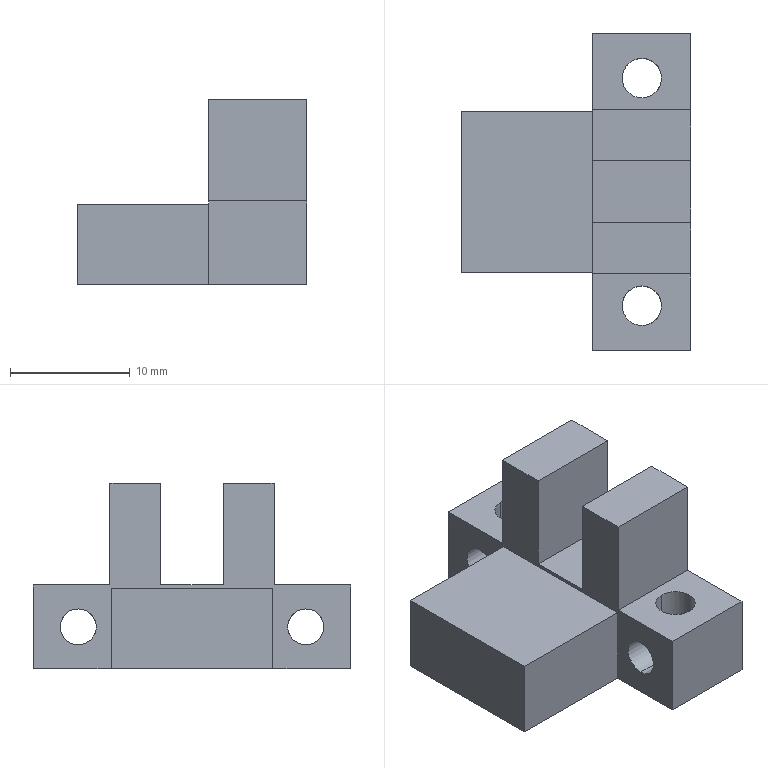Component | SolidWorks | 6G-OriginSwitch-1 | 1 solid | 30 faces | box 19.2 x 26.5 x 15.5 mm | volume 2914 mm3 | plane 18 | cylinder 12 | commonest cylinder face diameters 3 x8 3.3 x4
build123d program:
from build123d import *

# Parameters (mm, degrees)
SKETCH1_W           = 26.5
SKETCH1_H           = 15
BOSS_EXTRUDE1_DEPTH = 15.5
SKETCH2_W           = 5.2
SKETCH2_H           = 9.914
CUT_EXTRUDE1_DEPTH  = 26.314
SKETCH3_R           = 1.5
CUT_EXTRUDE2_DEPTH  = 26.314
FILLET1_R           = 0.5
SKETCH4_W           = 26.5
SKETCH4_H           = 3.4
CUT_EXTRUDE3_DEPTH  = 10
SKETCH5_W           = 13.5
SKETCH5_H           = 6.7
BOSS_EXTRUDE2_DEPTH = 11
SKETCH6_R           = 1.65
CUT_EXTRUDE4_DEPTH  = 22.813


with BuildPart() as part:
    # Sketch1 → Boss-Extrude1 (new body)
    with BuildSketch(Plane.XY):
        Rectangle(SKETCH1_W, SKETCH1_H)
    extrude(amount=BOSS_EXTRUDE1_DEPTH)

    # Sketch2 → Cut-Extrude1 (cut, through all)
    with BuildSketch(Plane.XZ.offset(7.5)):
        Polygon((-13.25, 7), (-6.85, 7), (-6.85, 16.914), (-14.613, 16.914), (-14.613, 7), align=None)
        Polygon((6.85, 16.914), (6.85, 7), (13.25, 7), (16.044, 7), (16.044, 16.914), align=None)
        with Locations((0, 11.957)):
            Rectangle(SKETCH2_W, SKETCH2_H)
    extrude(amount=-CUT_EXTRUDE1_DEPTH, mode=Mode.SUBTRACT)

    # Sketch3 → Cut-Extrude2 (cut, through all)
    with BuildSketch(Plane.XZ.offset(7.5)):
        with Locations(Location((-9.5, 3.5, 0), (0, 0, 270))):
            Circle(SKETCH3_R)
        with Locations(Location((9.5, 3.5, 0), (0, 0, 270))):
            Circle(SKETCH3_R)
    extrude(amount=-CUT_EXTRUDE2_DEPTH, mode=Mode.SUBTRACT)

    # Fillet1
    fillet1_edges = [part.edges().sort_by_distance(p)[0] for p in [
        (-13.25, -7.5, 3.5),
        (-13.25, 7.5, 3.5),
        (13.25, -7.5, 3.5),
        (13.25, 7.5, 3.5),
    ]]
    fillet(fillet1_edges, radius=FILLET1_R)

    # Sketch4 → Cut-Extrude3 (cut, symmetric)
    with BuildSketch(Plane.XY.offset(7)):
        with Locations((0, 5.8)):
            Rectangle(SKETCH4_W, SKETCH4_H)
        with Locations((0, -5.8)):
            Rectangle(SKETCH4_W, SKETCH4_H)
    extrude(amount=CUT_EXTRUDE3_DEPTH, both=True, mode=Mode.SUBTRACT)

    # Sketch5 → Boss-Extrude2 (add)
    with BuildSketch(Plane.XZ.offset(4.1)):
        with Locations((0, 3.35)):
            Rectangle(SKETCH5_W, SKETCH5_H)
    extrude(amount=BOSS_EXTRUDE2_DEPTH)

    # Sketch6 → Cut-Extrude4 (cut, through all)
    with BuildSketch(Plane.XY.offset(7)):
        with Locations((-9.5, 0)):
            Circle(SKETCH6_R)
        with Locations(Location((9.5, 0, 0), (0, 0, 180))):
            Circle(SKETCH6_R)
    extrude(amount=-CUT_EXTRUDE4_DEPTH, mode=Mode.SUBTRACT)


solid = part.part

# Placed as in the assembly
solid = solid.moved(Location((180.372, -79, 18.8), (0, 0, -90)))